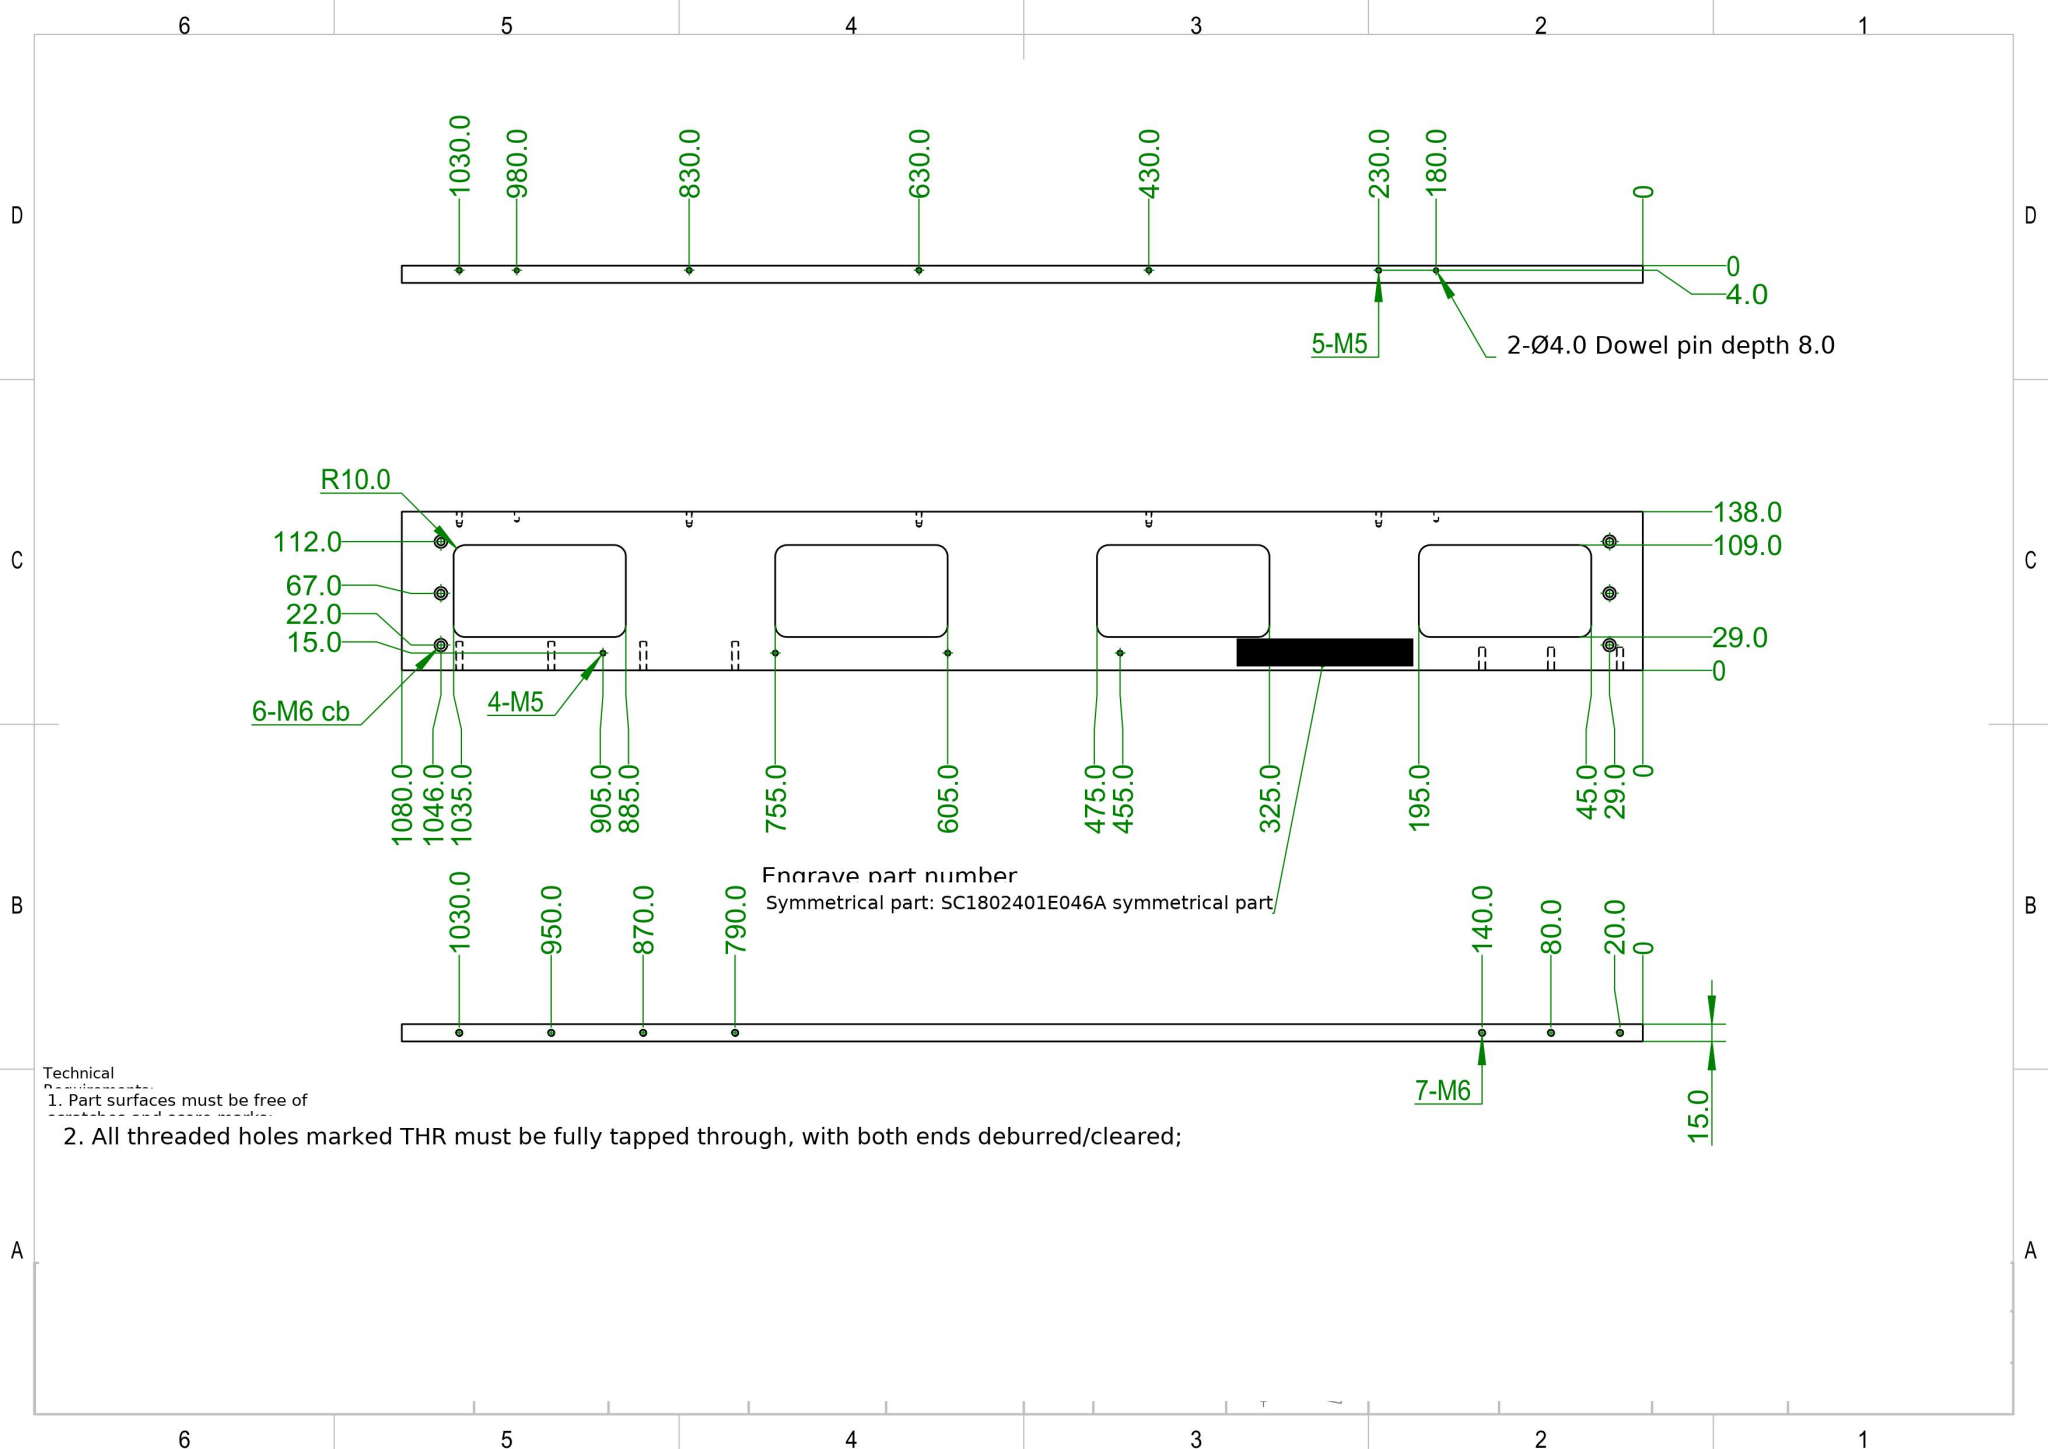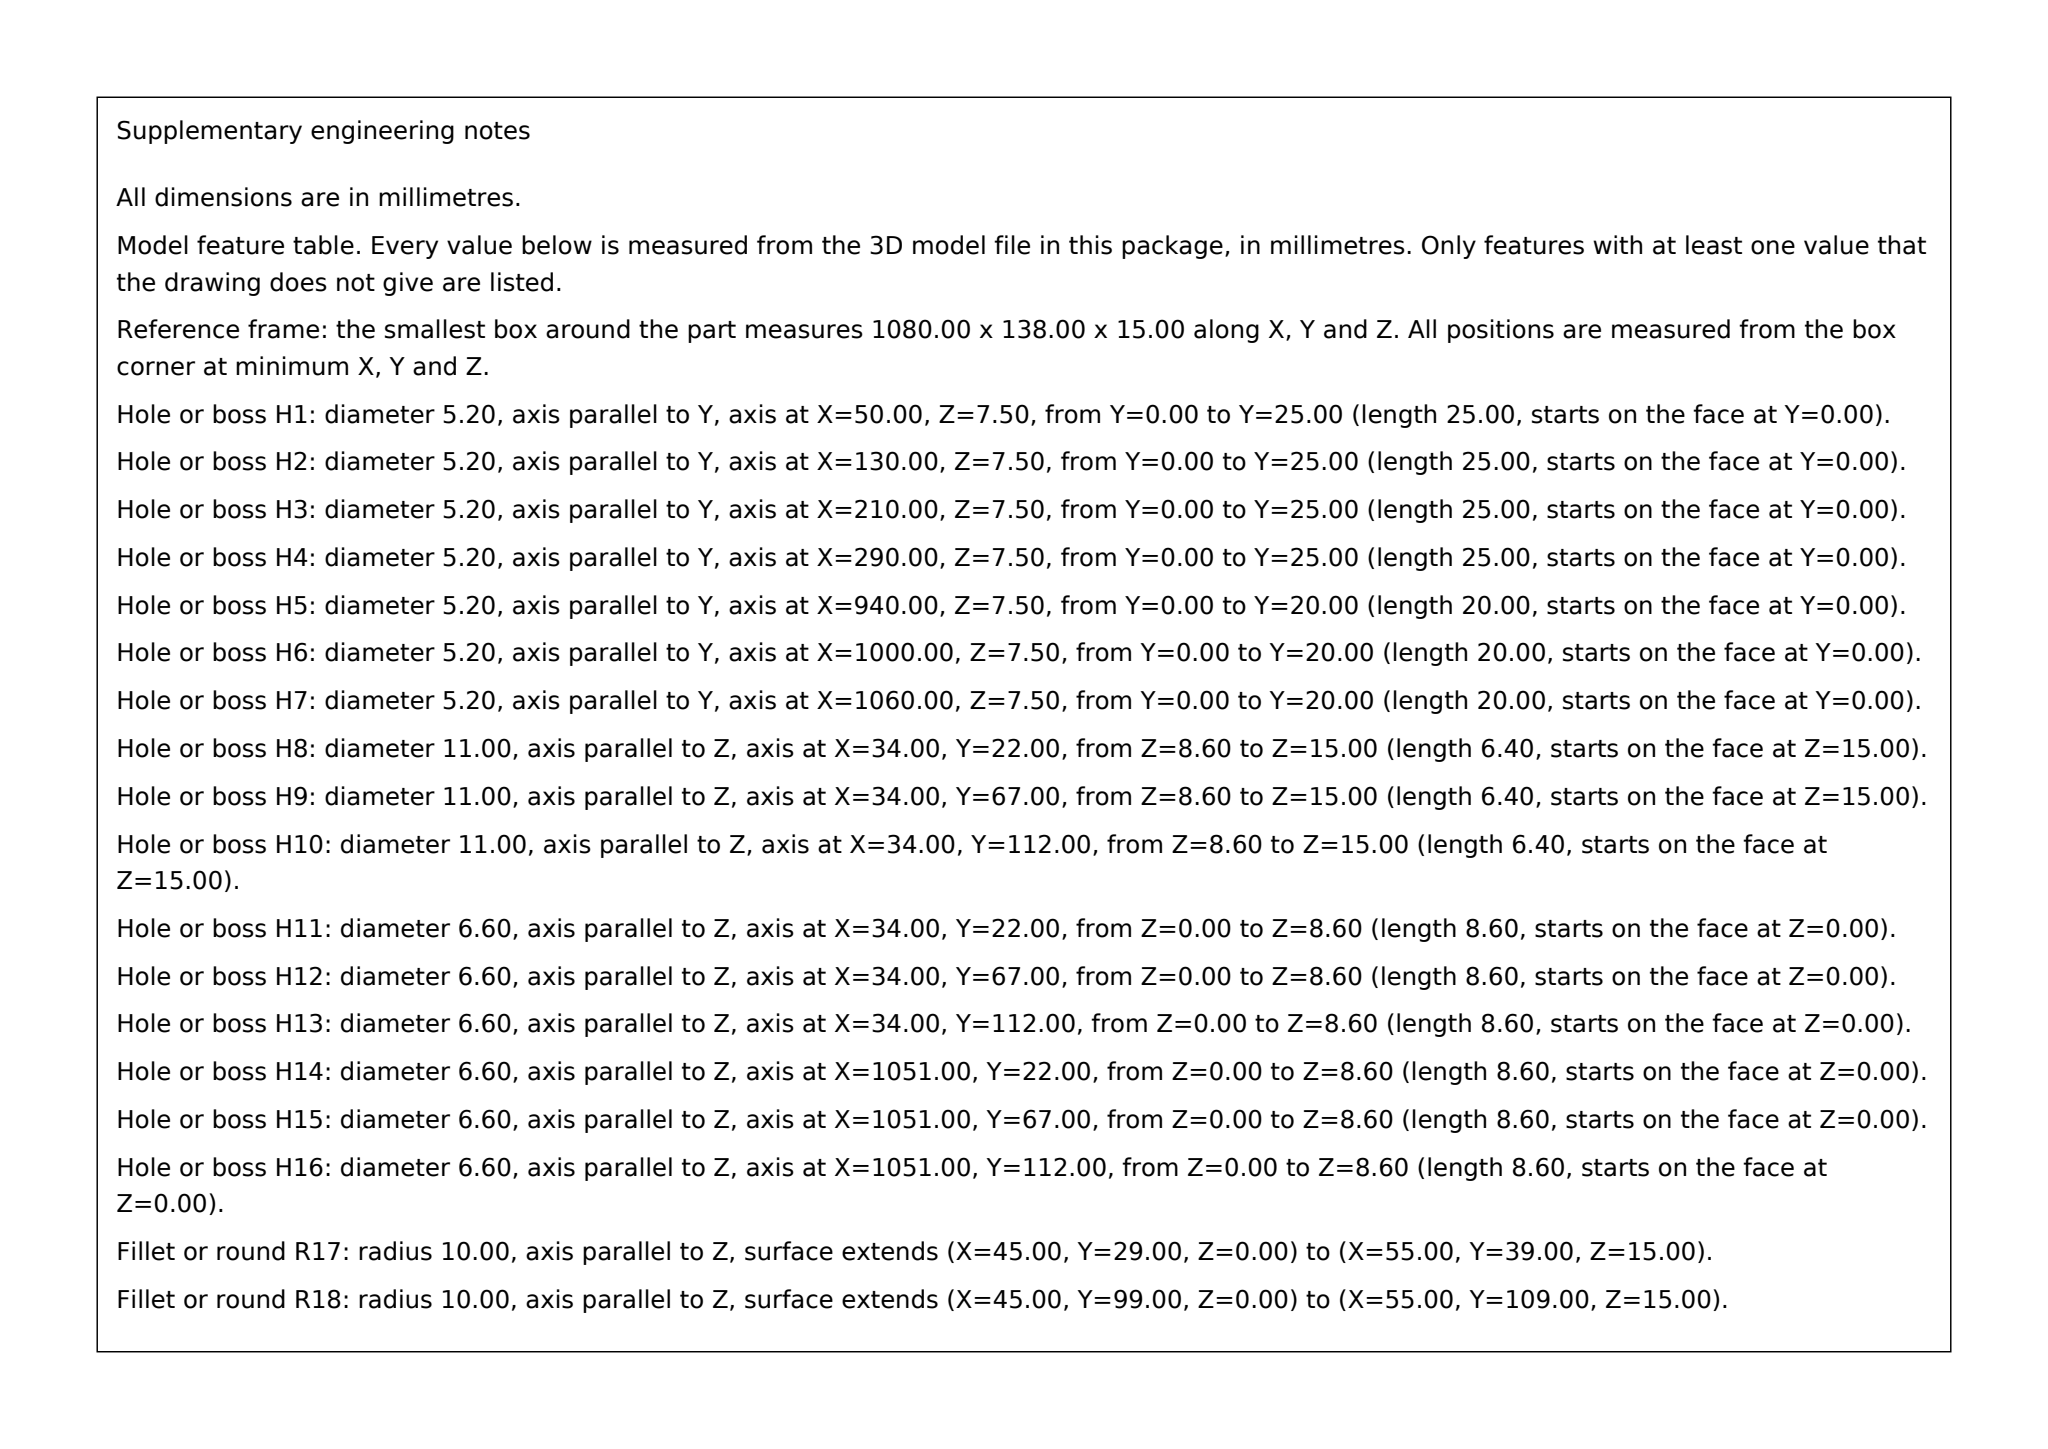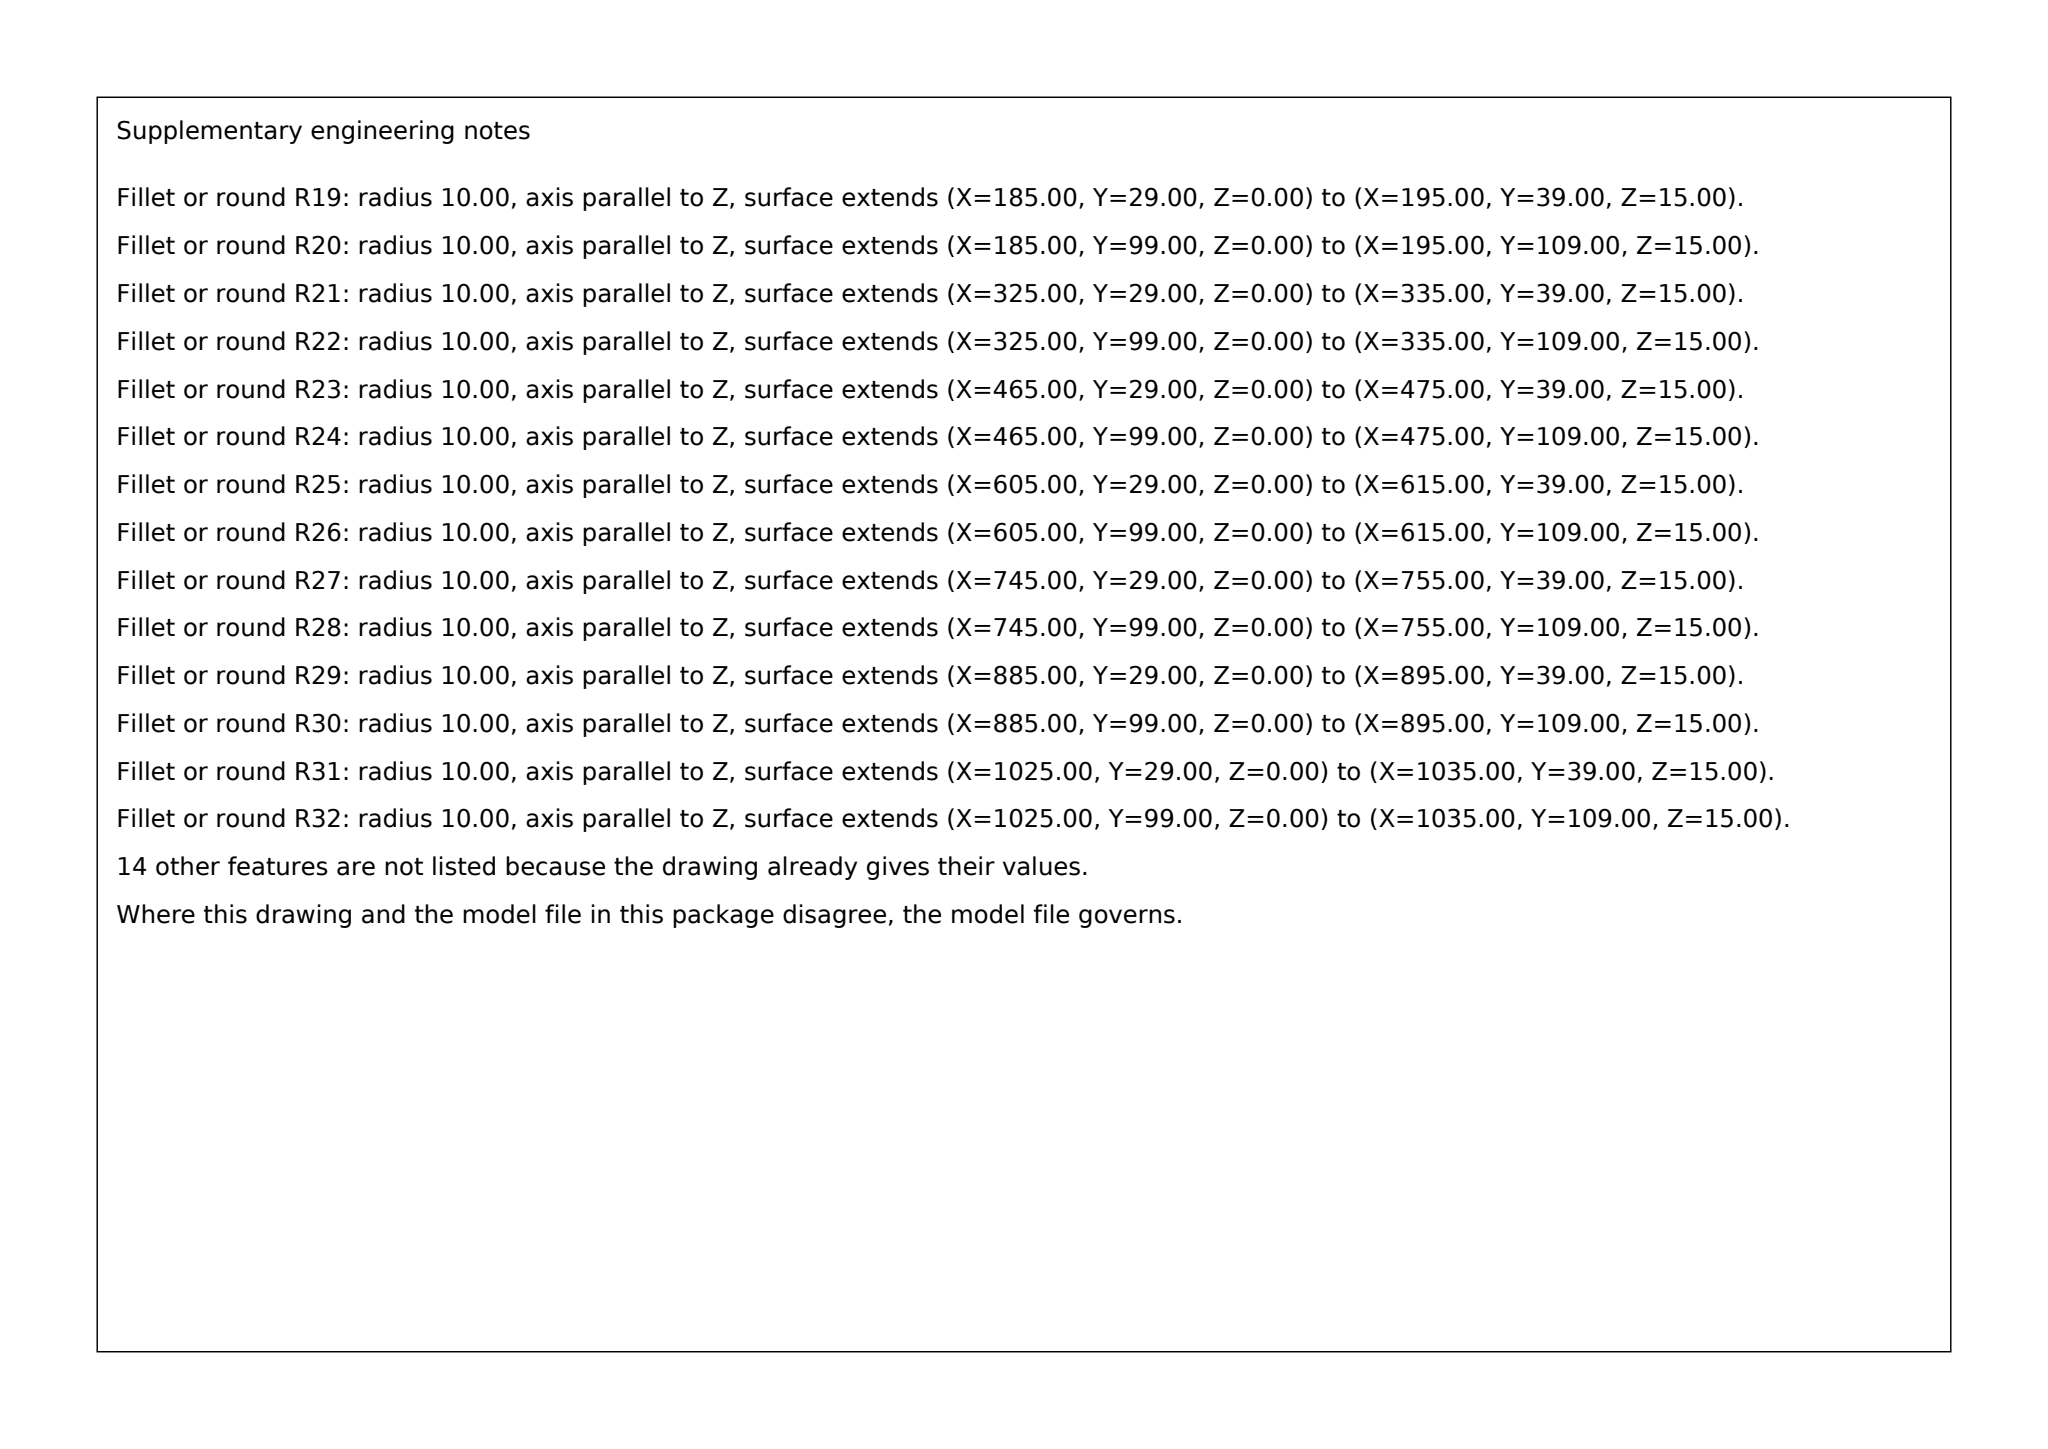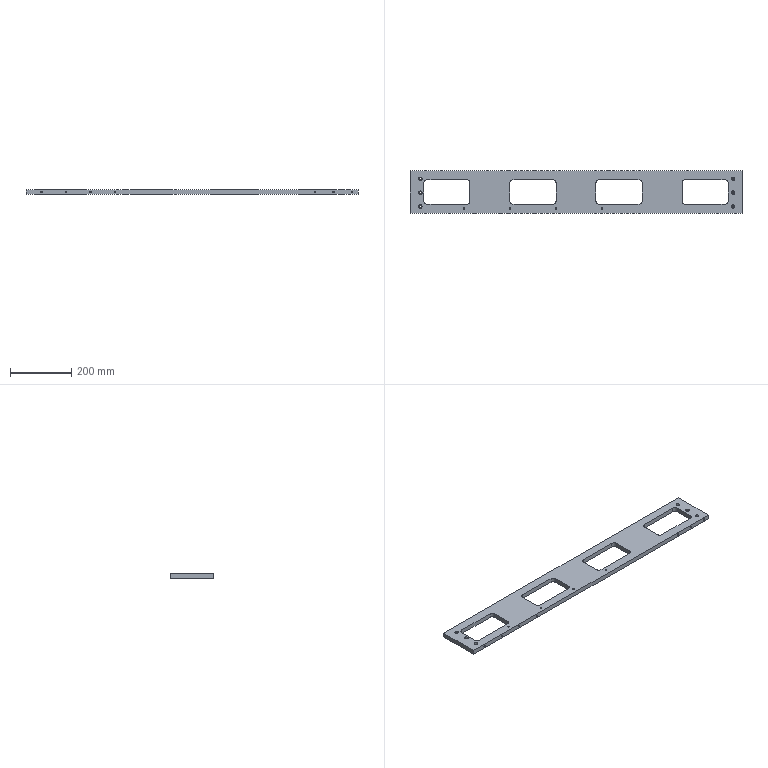Part | SolidWorks | mm | 1 solid | 125 faces | box 1080 x 138 x 15 mm | volume 1510007 mm3 | cylinder 76 | plane 35 | cone 14 | commonest cylinder face diameters 4.2 x18 20 x16 5.2 x14 11 x12 6.6 x12 4 x4
build123d program:
from build123d import *

# Parameters (mm, degrees)
SKETCH1_W                                       = 1080
SKETCH1_H                                       = 138
BOSS_EXTRUDE1_DEPTH                             = 7.5
SKETCH2_R                                       = 2.6
CUT_EXTRUDE1_DEPTH                              = 25
LPATTERN1_COUNT                                 = 4
LPATTERN1_PITCH                                 = 80
CUT_EXTRUDE2_DEPTH                              = 25
LPATTERN2_COUNT                                 = 4
LPATTERN2_PITCH                                 = 280
SKETCH5_R                                       = 2.6
CUT_EXTRUDE4_DEPTH                              = 20
M6_HEX_SOCKET_HEAD_CAP_SCREW_CBORE1_D           = 6.6
M6_HEX_SOCKET_HEAD_CAP_SCREW_CBORE1_CBORE_D     = 11
M6_HEX_SOCKET_HEAD_CAP_SCREW_CBORE1_CBORE_DEPTH = 6.4
M6_HEX_SOCKET_HEAD_CAP_SCREW_CBORE2_D           = 6.6
M6_HEX_SOCKET_HEAD_CAP_SCREW_CBORE2_CBORE_D     = 11
M6_HEX_SOCKET_HEAD_CAP_SCREW_CBORE2_CBORE_DEPTH = 6.4
M5_TAPPED_HOLE1_D                               = 4.2
M5_TAPPED_HOLE1_DEPTH                           = 12.4
M5_TAPPED_HOLE1_TIP                             = 1.262
SIZE_MM_DOWEL_PIN_HOLE_1_D                      = 4
SIZE_MM_DOWEL_PIN_HOLE_1_DEPTH                  = 8
SIZE_MM_DOWEL_PIN_HOLE_1_TIP                    = 1.202
M5_TAPPED_HOLE2_D                               = 4.2
LPATTERN3_COUNT                                 = 4
LPATTERN3_PITCH                                 = 150


with BuildPart() as part:
    # Sketch1 → Boss-Extrude1 (new, symmetric)
    with BuildSketch(Plane.XY):
        Rectangle(SKETCH1_W, SKETCH1_H)
    extrude(amount=BOSS_EXTRUDE1_DEPTH, both=True)

    # Sketch2 → Cut-Extrude1 (cut)
    with BuildSketch(Plane.XZ.offset(69)):
        with Locations(Location((-490, 0, 0), (0, 0, 270))):
            Circle(SKETCH2_R)
    cut_extrude1 = extrude(amount=-CUT_EXTRUDE1_DEPTH, mode=Mode.SUBTRACT)

    # LPattern1: Cut-Extrude1 ×4
    with Locations(*[(i * LPATTERN1_PITCH, 0, 0) for i in range(1, LPATTERN1_COUNT)]):
        add(cut_extrude1, mode=Mode.SUBTRACT)

    # Sketch3 → Cut-Extrude2 (cut)
    with BuildSketch(Plane.XY.offset(7.5)):
        with BuildLine():
            Line((-485, 40), (-355, 40))
            ThreePointArc((-355, 40), (-347.929, 37.071), (-345, 30))
            Line((-345, 30), (-345, -30))
            ThreePointArc((-345, -30), (-347.929, -37.071), (-355, -40))
            Line((-355, -40), (-485, -40))
            ThreePointArc((-485, -40), (-492.071, -37.071), (-495, -30))
            Line((-495, -30), (-495, 30))
            ThreePointArc((-495, 30), (-492.071, 37.071), (-485, 40))
        make_face()
    cut_extrude2 = extrude(amount=-CUT_EXTRUDE2_DEPTH, mode=Mode.SUBTRACT)

    # LPattern2: Cut-Extrude2 ×4
    with Locations(*[(i * LPATTERN2_PITCH, 0, 0) for i in range(1, LPATTERN2_COUNT)]):
        add(cut_extrude2, mode=Mode.SUBTRACT)

    # Sketch5 → Cut-Extrude4 (cut)
    with BuildSketch(Plane.XZ.offset(69)):
        with Locations(Location((400, 0, 0), (0, 0, 270))):
            Circle(SKETCH5_R)
        with Locations(Location((460, 0, 0), (0, 0, 270))):
            Circle(SKETCH5_R)
        with Locations(Location((520, 0, 0), (0, 0, 270))):
            Circle(SKETCH5_R)
    extrude(amount=-CUT_EXTRUDE4_DEPTH, mode=Mode.SUBTRACT)

    # M6 Hex Socket Head Cap Screw CBORE1 (through all)
    with Locations(Plane.XY.offset(7.5)):
        with Locations((511, 43), (511, -2), (511, -47)):
            CounterBoreHole(M6_HEX_SOCKET_HEAD_CAP_SCREW_CBORE1_D / 2, M6_HEX_SOCKET_HEAD_CAP_SCREW_CBORE1_CBORE_D / 2, M6_HEX_SOCKET_HEAD_CAP_SCREW_CBORE1_CBORE_DEPTH)

    # M6 Hex Socket Head Cap Screw CBORE2 (through all)
    with Locations(Plane.XY.offset(7.5)):
        with Locations((-506, 43), (-506, -2), (-506, -47)):
            CounterBoreHole(M6_HEX_SOCKET_HEAD_CAP_SCREW_CBORE2_D / 2, M6_HEX_SOCKET_HEAD_CAP_SCREW_CBORE2_CBORE_D / 2, M6_HEX_SOCKET_HEAD_CAP_SCREW_CBORE2_CBORE_DEPTH)

    # M5 Tapped Hole1
    with Locations(Plane(origin=(0, 69, 0), x_dir=(1, 0, 0), z_dir=(0, 1, 0))):
        with Locations((-490, 3.5), (-290, 3.5), (-90, 3.5), (110, 3.5), (310, 3.5)):
            Hole(M5_TAPPED_HOLE1_D / 2, depth=M5_TAPPED_HOLE1_DEPTH)
            with Locations((0, 0, -(M5_TAPPED_HOLE1_DEPTH + M5_TAPPED_HOLE1_TIP / 2))):  # 118° drill point
                Cone(0, M5_TAPPED_HOLE1_D / 2, M5_TAPPED_HOLE1_TIP, mode=Mode.SUBTRACT)

    # Size mm Dowel Pin Hole 1
    with Locations(Plane(origin=(0, 69, 0), x_dir=(1, 0, 0), z_dir=(0, 1, 0))):
        with Locations((-440, 3.5), (360, 3.5)):
            Hole(SIZE_MM_DOWEL_PIN_HOLE_1_D / 2, depth=SIZE_MM_DOWEL_PIN_HOLE_1_DEPTH)
            with Locations((0, 0, -(SIZE_MM_DOWEL_PIN_HOLE_1_DEPTH + SIZE_MM_DOWEL_PIN_HOLE_1_TIP / 2))):  # 118° drill point
                Cone(0, SIZE_MM_DOWEL_PIN_HOLE_1_D / 2, SIZE_MM_DOWEL_PIN_HOLE_1_TIP, mode=Mode.SUBTRACT)

    # M5 Tapped Hole2 (through all)
    with Locations(Plane.XY.offset(7.5)):
        with Locations((85, -54)):
            m5_tapped_hole2 = Hole(M5_TAPPED_HOLE2_D / 2)

    # LPattern3: M5 Tapped Hole2 ×4
    with Locations(*[(-i * LPATTERN3_PITCH, 0, 0) for i in range(1, LPATTERN3_COUNT)]):
        add(m5_tapped_hole2, mode=Mode.SUBTRACT)


solid = part.part